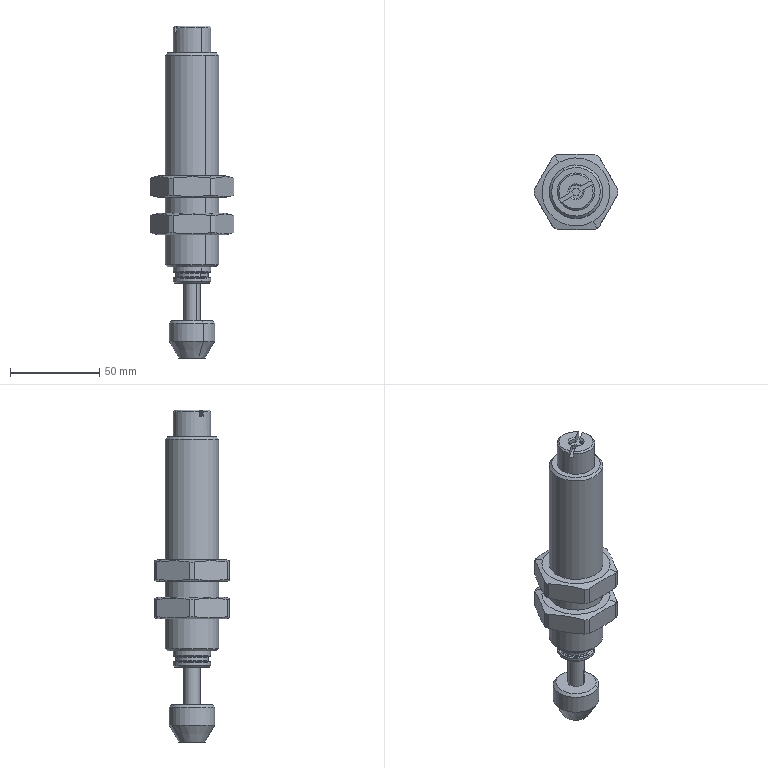Component | SolidWorks | HydraulicBufferACA1007-1AIRTAC-1 | 3 solids | 107 faces | volume 121444 mm3 | plane 37 | cylinder 35 | cone 27 | spline 8 | commonest cylinder face diameters 47.059 x14 30 x6 21 x6 7.377 x3 18 x2 9 x2 25.5 x2